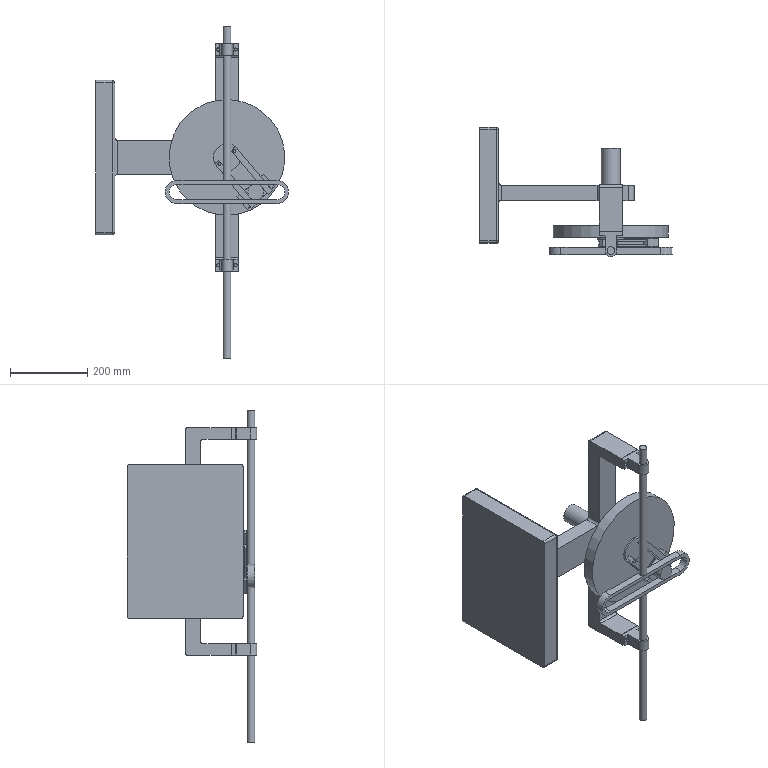Assembly | NX | mm | 14 component files | 15 solids | 165 faces | box 500.71 x 335.49 x 861 mm | volume 11840572 mm3 | plane 109 | cylinder 52 | sphere 4 | commonest cylinder face diameters 12 x18 8 x8 6 x5 20 x4 30 x3 41 x3 42 x2 50 x2
Bill of materials:
unnamed part 1 | 1 |  | Bracket-like part: a thin rectangular plate with a straight rectangular arm sticking out from its face. At the arm's far end is a flat C-shaped strip with short return flanges at both ends, plus a small rounded tab with a round through-hole where the arm meets the C-strip.
unnamed part 2 | 1 |  | Rectangular block with a stepped internal channel. One side view shows two solid end portions joined by a thin web along one edge, with a stepped (T-like) gap between them. The other side view shows a C-shaped section with stepped inner shoulders.
unnamed part 3 | 2 |  | Long, slender plain cylindrical rod with flat ends.
unnamed part 4 | 1 |  | Thin flat circular disc with two small round through-holes placed diametrically opposite each other near the rim.
unnamed part 5 | 1 |  | Solid plain cylinder, with length roughly equal to diameter.
unnamed part 6 | 1 |  | Thin-walled, open obround (stadium-shaped) ring or loop band with uniform wall thickness and short height.
unnamed part 7 | 2 |  | T-shaped bracket: a rectangular flange plate with two round through-holes, joined to a perpendicular web. The web ends in a rounded lug with a large round through-bore.
unnamed part 8 | 2 |  | Long rectangular bar with one small round through-hole near one end and a small rectangular notch or slot at that same end.
unnamed part 9 | 1 |  | Solid flat block with an obround (stadium) cross-section, rounded at both ends and of moderate uniform thickness.
unnamed part 10 | 1 |  | Stepped cylindrical shaft or pin: a long main diameter with a shorter, smaller-diameter section at one end. A small notch or flat sits near the edge of the smaller end.
unnamed part 11 | 1 |  | Thin flat circular disc with a central round bore and a very small notch at the edge of the bore.
Mates:
1. touch align | kama 1 face | model2 1 face
2. touch align | kama 1 face | model2 1 face
3. distance | kama 1 edge | model2 1 edge
4. touch align | model1 1 face | model2 1 face
5. touch align | model2 1 edge | model1 1 edge
6. touch align | kama 1 face | model1 1 face
7. touch align | model5 1 face | model7 1 face
8. touch align | model5 1 face | model7 2 face
9. touch align | model5 1 face | model7 1 face
10. touch align | model5 1 face | model7 2 face
11. touch align | model4 1 face | model5 1 face
12. distance | model4 1 edge | model5 1 edge
13. touch align | model4 1 face | model7 1 face
14. touch align | model4 1 face | model3 1 face
15. touch align | model3 1 face | model4 1 face
16. distance | model3 1 face | model7 2 face
17. touch align | sirt 1 face | model2 1 face
18. fix | sirt 1 component
19. touch align | d 2 face | yatak 2 face
20. touch align | d 1 face | yatak 1 face
21. touch align | d 1 face | model3 1 face
22. touch align | d 2 face | model3 1 face
23. touch align | d 1 edge | model3 1 edge
24. fix | yatak 1 component
25. fix | yatak 2 component
26. distance | model3 1 face | sirt 1 face
27. touch align | model8 1 face | model2 1 face
28. touch align | model8 1 face | model1 1 face
29. distance | model2 1 face | model4 1 face
30. parallel | model7 1 face | model7 2 face
31. touch align | model7 2 face | model8 1 face
32. touch align | model7 1 face | model8 1 face